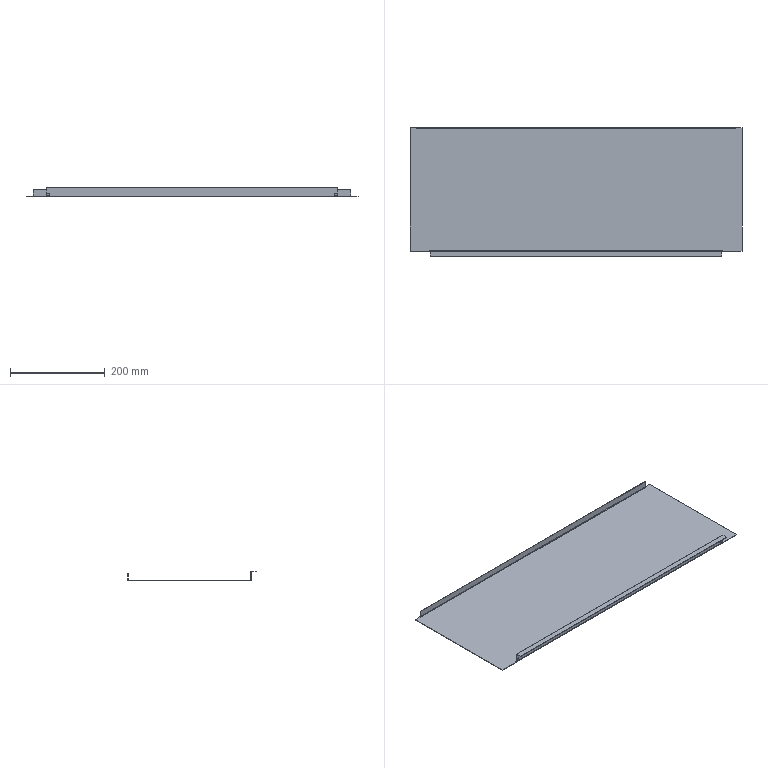Component | SolidWorks | CCQ-1.1-4SideUpperPlate1-3 | 1 solid | 50 faces | volume 209553 mm3 | plane 40 | cylinder 10 | commonest cylinder face diameters 6 x4 3.473 x3 1.473 x3 | material 304